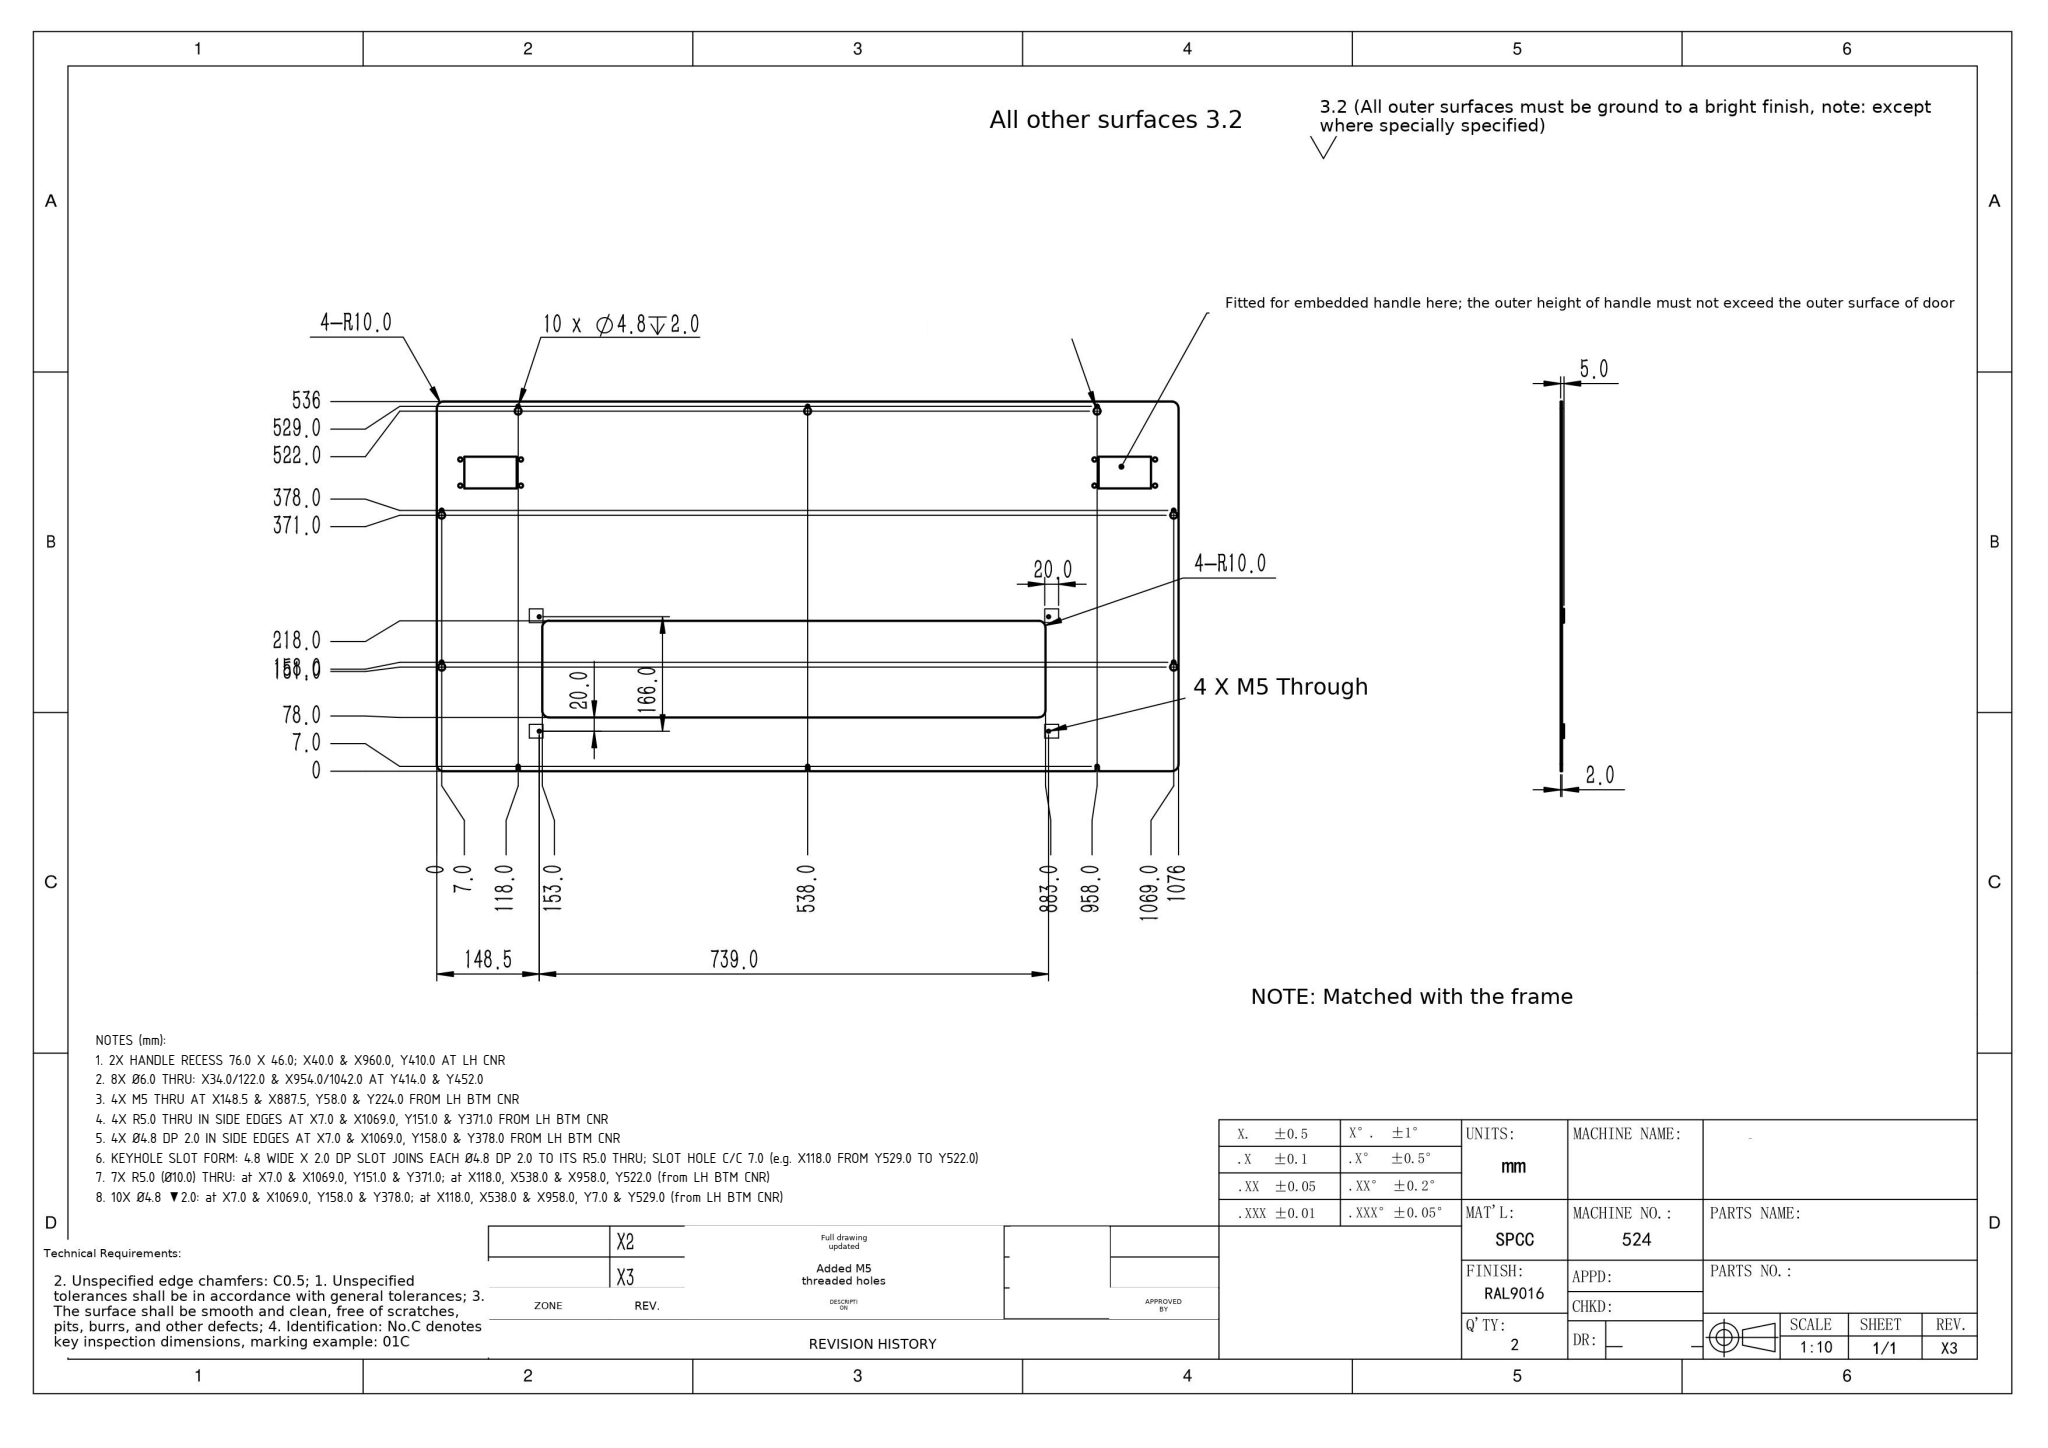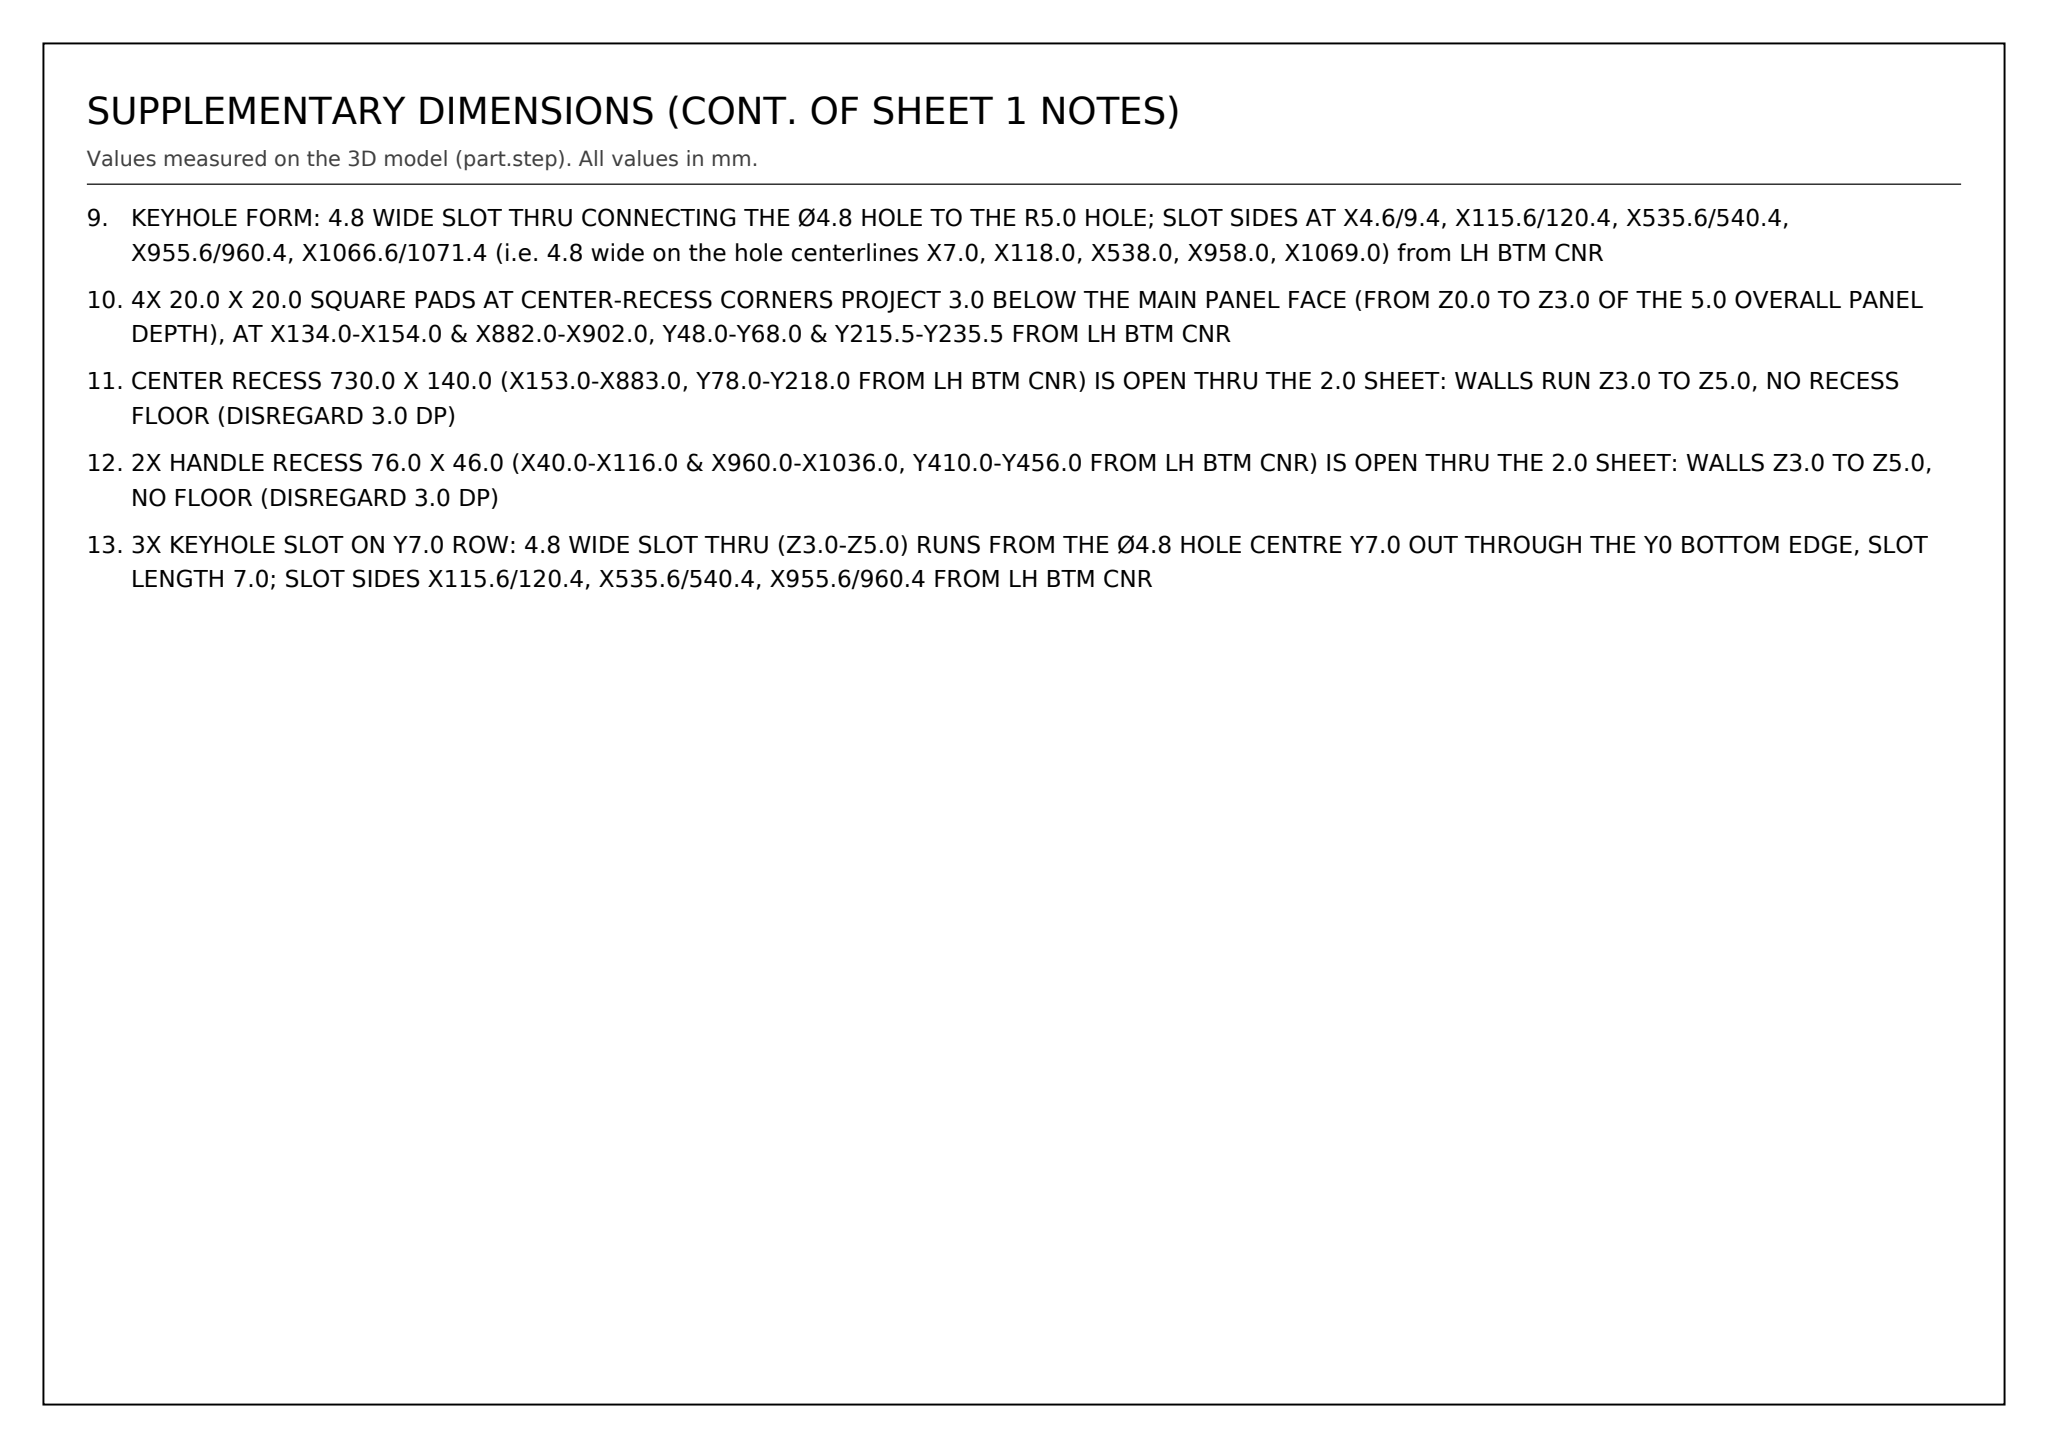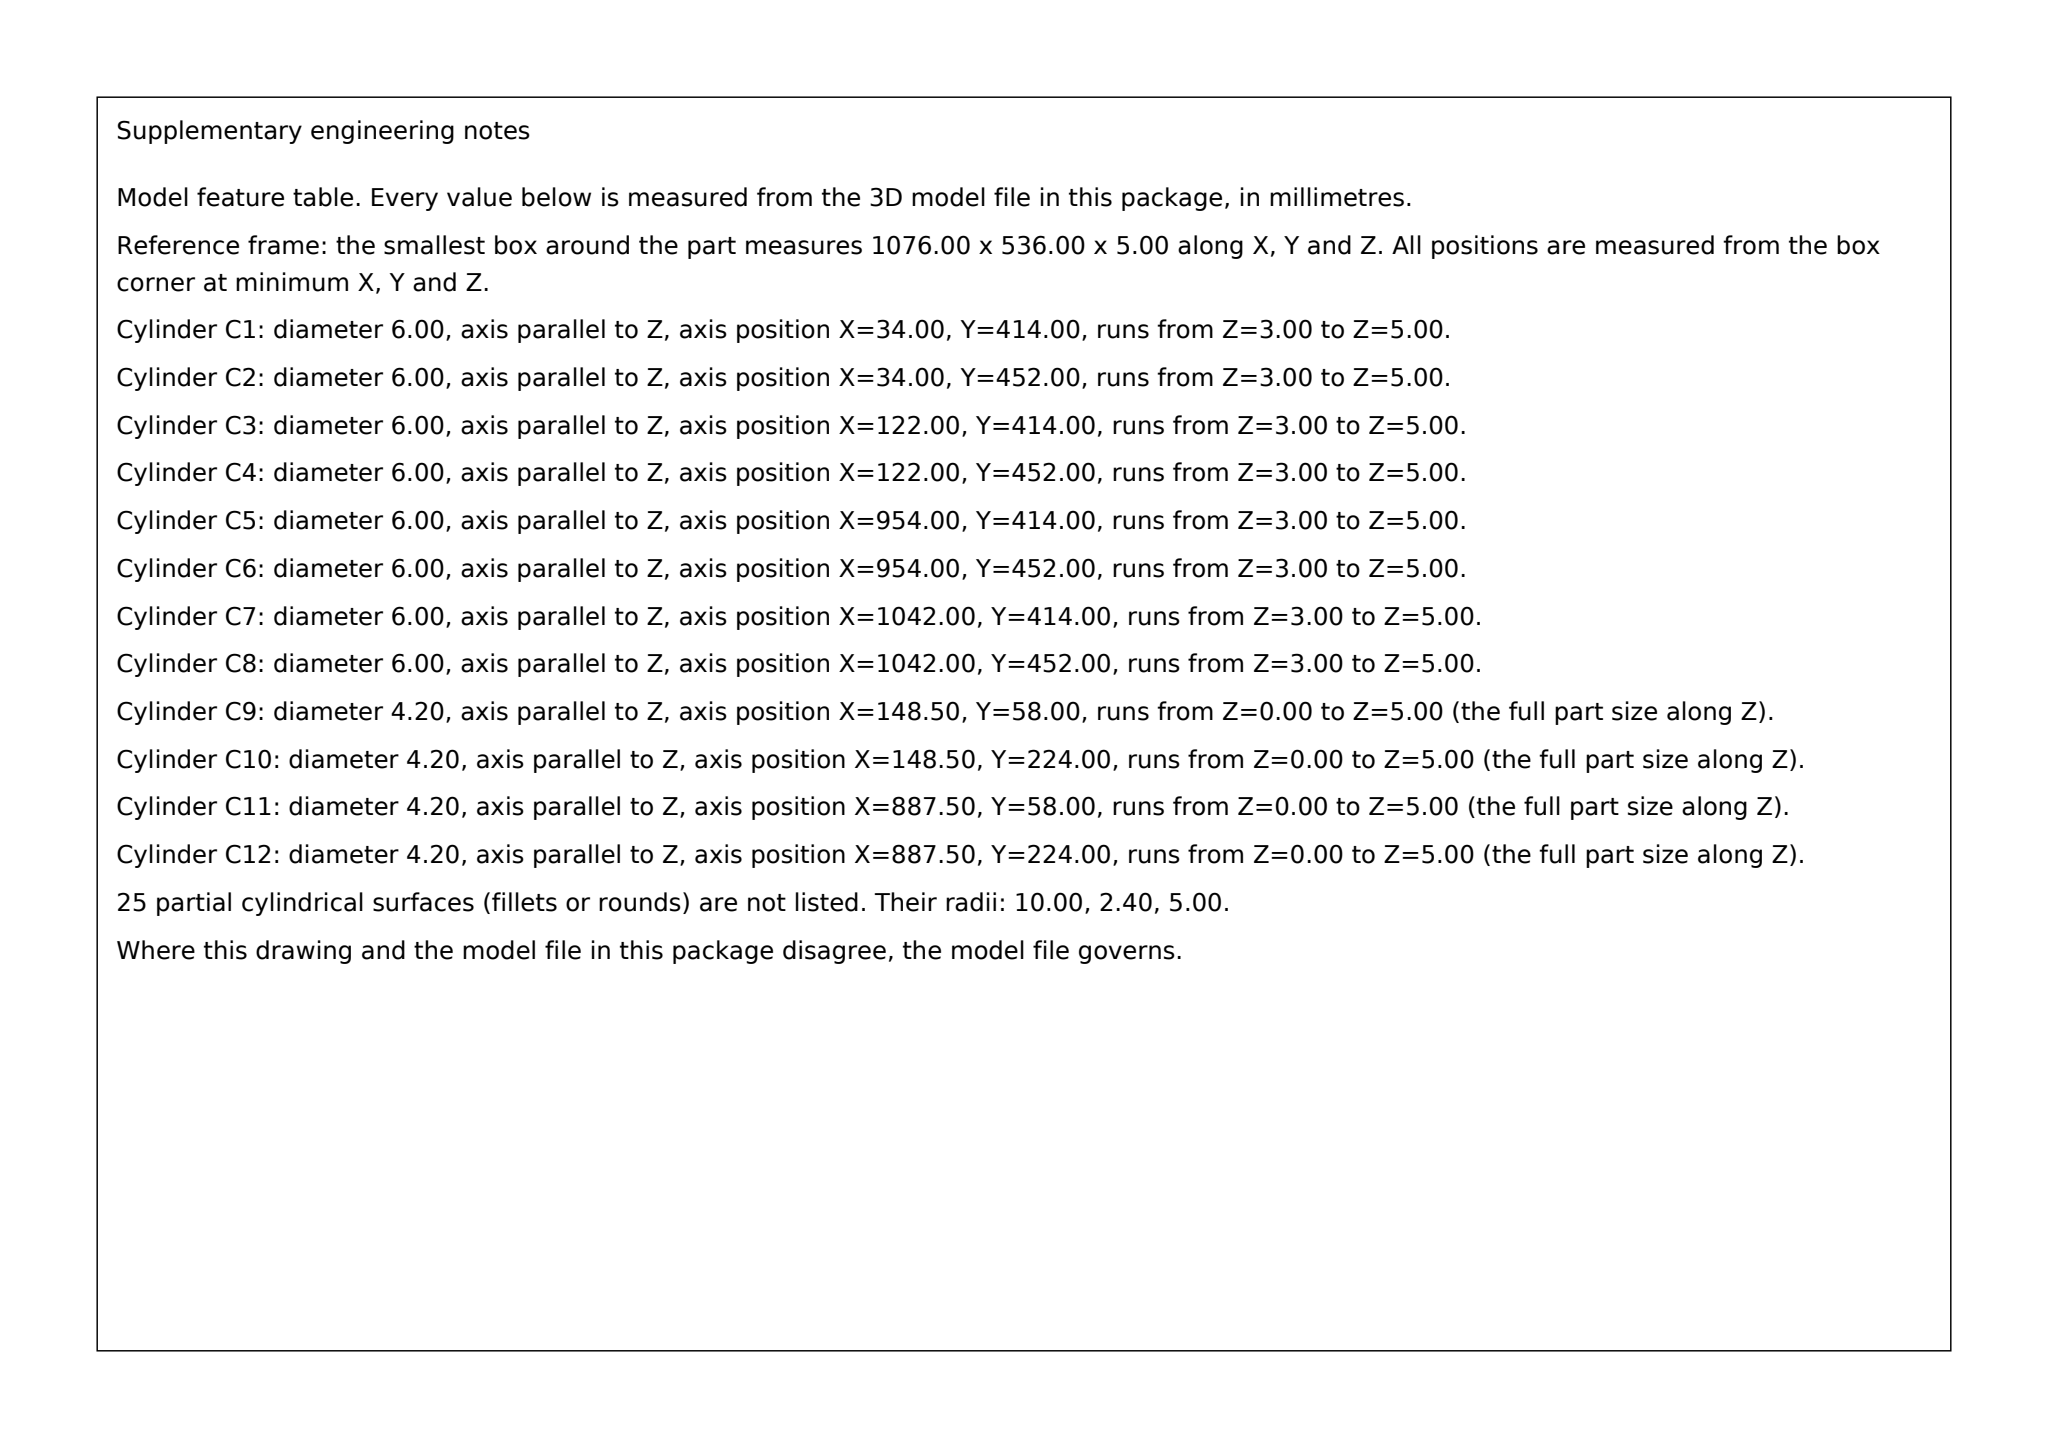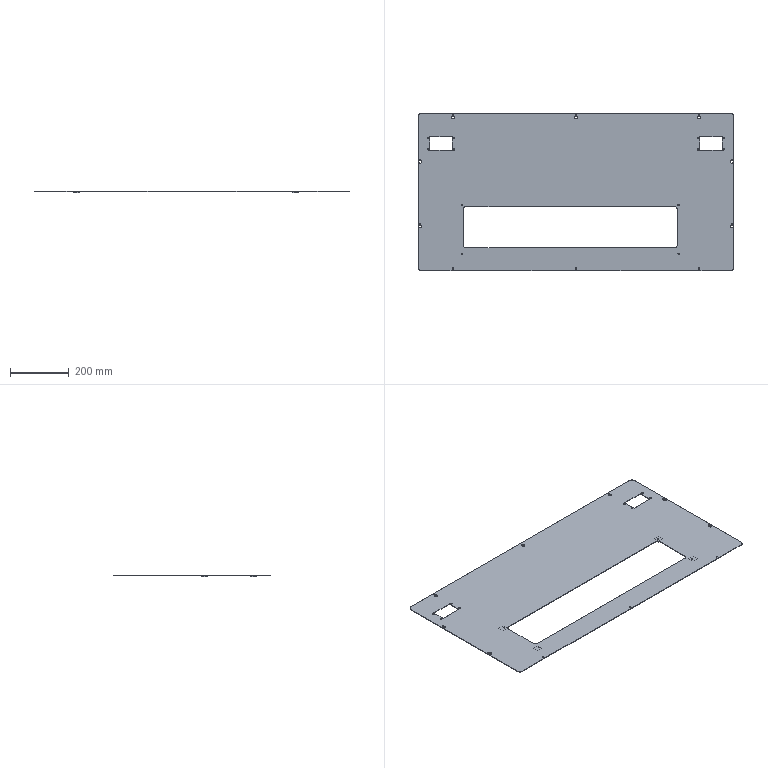Part | SolidWorks | mm | 1 solid | 124 faces | box 1076 x 536 x 5 mm | volume 937529 mm3 | cylinder 63 | plane 61 | commonest cylinder face diameters 10 x21 6 x16 4.8 x10 4.2 x8 20 x8
Drawing notes:
2X HANDLE RECESS 76.0 X 46.0; X40.0 & X960.0, Y410.0 AT LH CNR | from the solid: x-planes 40.0/116.0 & 960.0/1036.0 (76 wide), y-planes 410.0/456.0 (46 high), 2 off
8X Ø6.0 THRU: X34.0/122.0 & X954.0/1042.0 AT Y414.0 & Y452.0 | from the solid: Ø6.0 z-cylinders at (34,414)(34,452)(122,414)(122,452)(954,414)(954,452)(1042,414)(1042,452), len 2.0 = thru
4X M5 THRU AT X148.5 & X887.5, Y58.0 & Y224.0 FROM LH BTM CNR | from the solid: Ø4.2 z-cylinders len 5.0 (full bbox depth) at (148.5,58)(148.5,224)(887.5,58)(887.5,224)
4X R5.0 THRU IN SIDE EDGES AT X7.0 & X1069.0, Y151.0 & Y371.0 FROM LH BTM CNR | from the solid: cylinders dia 10.0 axis z at (7.0,151.0), (7.0,371.0), (1069.0,151.0), (1069.0,371.0), length 2.0
4X Ø4.8 DP 2.0 IN SIDE EDGES AT X7.0 & X1069.0, Y158.0 & Y378.0 FROM LH BTM CNR | from the solid: cylinders dia 4.8 axis z at (7.0,158.0), (7.0,378.0), (1069.0,158.0), (1069.0,378.0), length 2.0
KEYHOLE SLOT FORM: 4.8 WIDE X 2.0 DP SLOT JOINS EACH Ø4.8 DP 2.0 TO ITS R5.0 THRU; SLOT HOLE C/C 7.0 (e.g. X118.0 FROM Y529.0 TO Y522.0) | from the solid: x-plane pairs 4.6/9.4, 115.6/120.4, 535.6/540.4, 955.6/960.4, 1066.6/1071.4 (4.8 apart) with dia 4.8 and dia 10.0 cylinder centres 7.0 apart
7X R5.0 (Ø10.0) THRU: at X7.0 & X1069.0, Y151.0 & Y371.0; at X118.0, X538.0 & X958.0, Y522.0 (from LH BTM CNR) | from the solid: cylinders dia 10.0 axis z at [7.0,151.0], [7.0,371.0], [1069.0,151.0], [1069.0,371.0], [118.0,522.0], [538.0,522.0], [958.0,522.0]
10X Ø4.8 ▼2.0: at X7.0 & X1069.0, Y158.0 & Y378.0; at X118.0, X538.0 & X958.0, Y7.0 & Y529.0 (from LH BTM CNR) | from the solid: cylinders dia 4.8 axis z at [7.0,158.0], [7.0,378.0], [1069.0,158.0], [1069.0,378.0], [118.0,7.0], [118.0,529.0], [538.0,7.0], [538.0,529.0], [958.0,7.0], [958.0,529.0]
KEYHOLE FORM: 4.8 WIDE SLOT THRU CONNECTING THE Ø4.8 HOLE TO THE R5.0 HOLE; SLOT SIDES AT X4.6/9.4, X115.6/120.4, X535.6/540.4, X955.6/960.4, X1066.6/1071.4 (i.e. 4.8 wide on the hole centerlines X7.0, X118.0, X538.0, X958.0, X1069.0) from LH BTM CNR | from the solid: axis_planes x 4.6, 9.4, 115.6, 120.4, 535.6, 540.4, 955.6, 960.4, 1066.6, 1071.4 (pairs 4.8 apart) with dia 4.8 / dia 10.0 cylinders on those centers
4X 20.0 X 20.0 SQUARE PADS AT CENTER-RECESS CORNERS PROJECT 3.0 BELOW THE MAIN PANEL FACE (FROM Z0.0 TO Z3.0 OF THE 5.0 OVERALL PANEL DEPTH), AT X134.0-X154.0 & X882.0-X902.0, Y48.0-Y68.0 & Y215.5-Y235.5 FROM LH BTM CNR | from the solid: axis_planes: z-normal faces at z=0.0 with extents x[134.0,154.0]/[882.0,902.0] and y[48.0,68.0]/[215.5,235.5]; x- and y-normal side faces of these pads span z[0.0,3.0]; main panel face plane z=3.0 spans x[0,1076] y[0,536]; bbox_xyz z=5.0
CENTER RECESS 730.0 X 140.0 (X153.0-X883.0, Y78.0-Y218.0 FROM LH BTM CNR) IS OPEN THRU THE 2.0 SHEET: WALLS RUN Z3.0 TO Z5.0, NO RECESS FLOOR (DISREGARD 3.0 DP) | from the solid: axis_planes x=153.0 & x=883.0 extent y[88,208] z[3.0,5.0]; y=78.0 & y=218.0 extent x[163,873] z[3.0,5.0]; only z-plane present is z=3.0 over full 1076x536 (no floor plane inside recess)
2X HANDLE RECESS 76.0 X 46.0 (X40.0-X116.0 & X960.0-X1036.0, Y410.0-Y456.0 FROM LH BTM CNR) IS OPEN THRU THE 2.0 SHEET: WALLS Z3.0 TO Z5.0, NO FLOOR (DISREGARD 3.0 DP) | from the solid: axis_planes x=40.0/116.0/960.0/1036.0 extent y[410.0,456.0] z[3.0,5.0] and y=410.0/456.0 extent x[40,116] & x[960,1036] z[3.0,5.0]; no z-plane floor in recess
3X KEYHOLE SLOT ON Y7.0 ROW: 4.8 WIDE SLOT THRU (Z3.0-Z5.0) RUNS FROM THE Ø4.8 HOLE CENTRE Y7.0 OUT THROUGH THE Y0 BOTTOM EDGE, SLOT LENGTH 7.0; SLOT SIDES X115.6/120.4, X535.6/540.4, X955.6/960.4 FROM LH BTM CNR | from the solid: axis_planes x=115.6, 120.4, 535.6, 540.4, 955.6, 960.4 each extent y[0.0,7.0] z[3.0,5.0]; y=0.0 face broken into x[10,115.6], [120.4,535.6], [540.4,955.6], [960.4,1066]